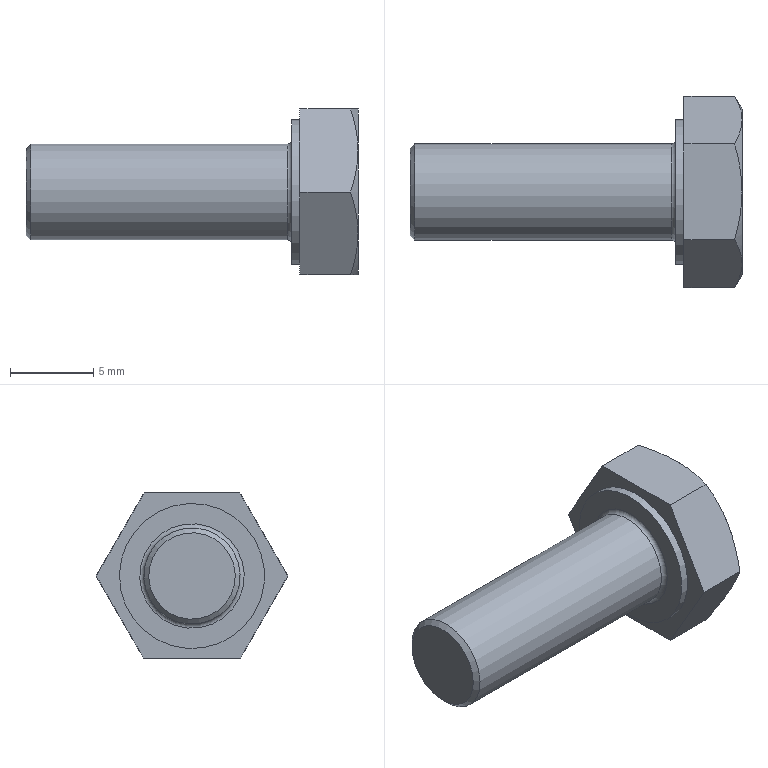Component | NX | GB-T5782-2000_M6X16_10 | 1 solid | 20 faces | volume 754 mm3 | plane 10 | cone 7 | cylinder 2 | torus 1 | commonest cylinder face diameters 8.74 x1 5.795 x1